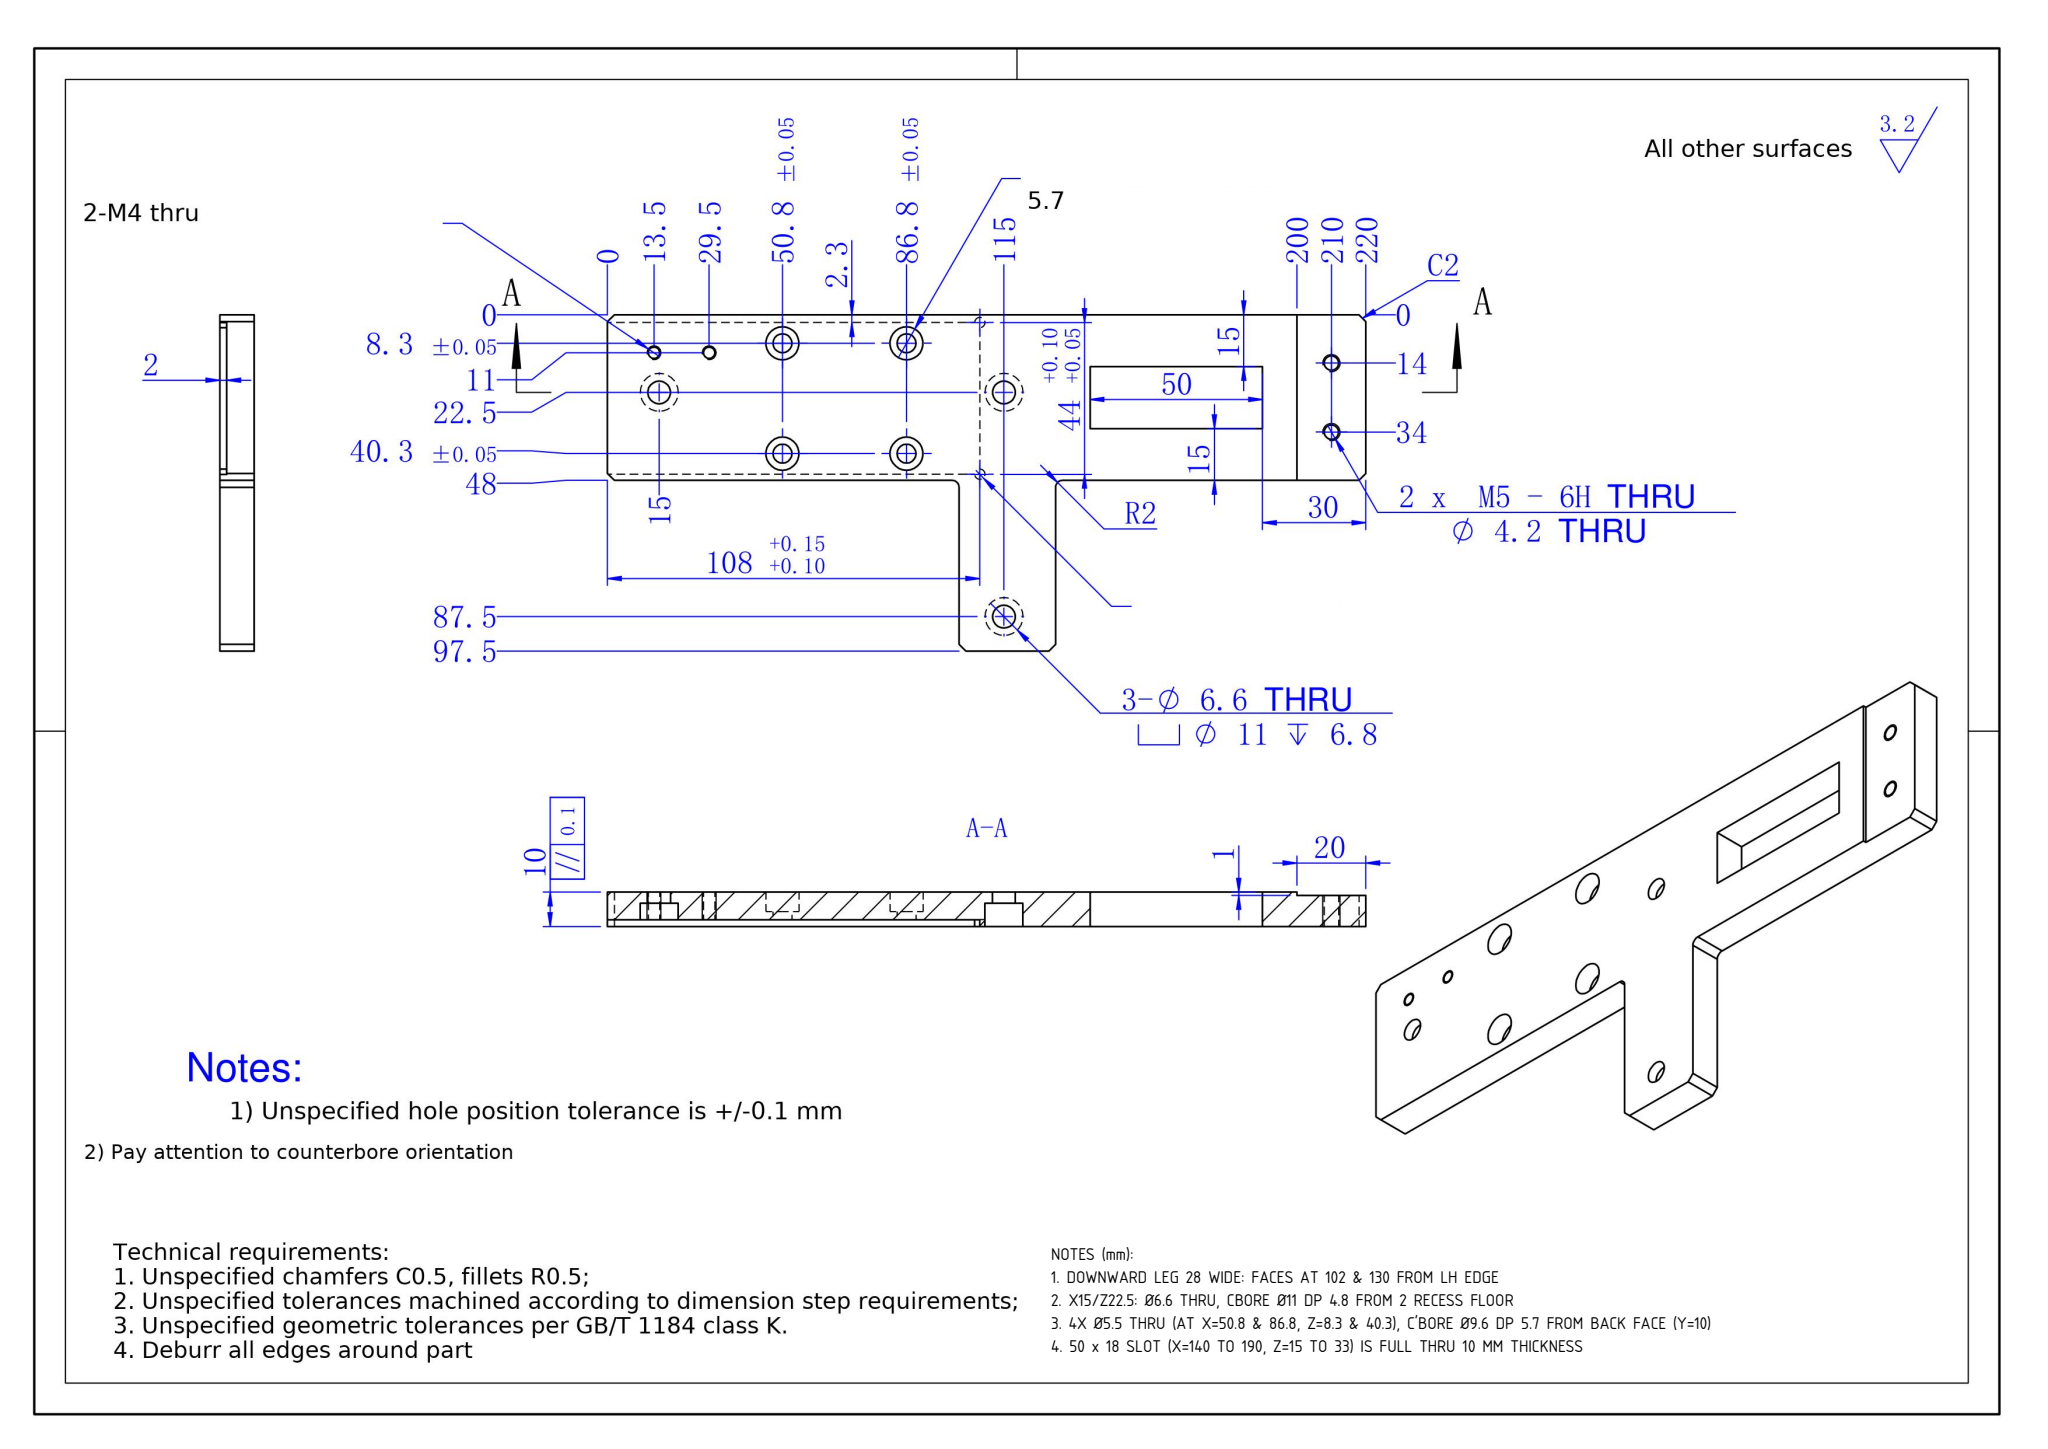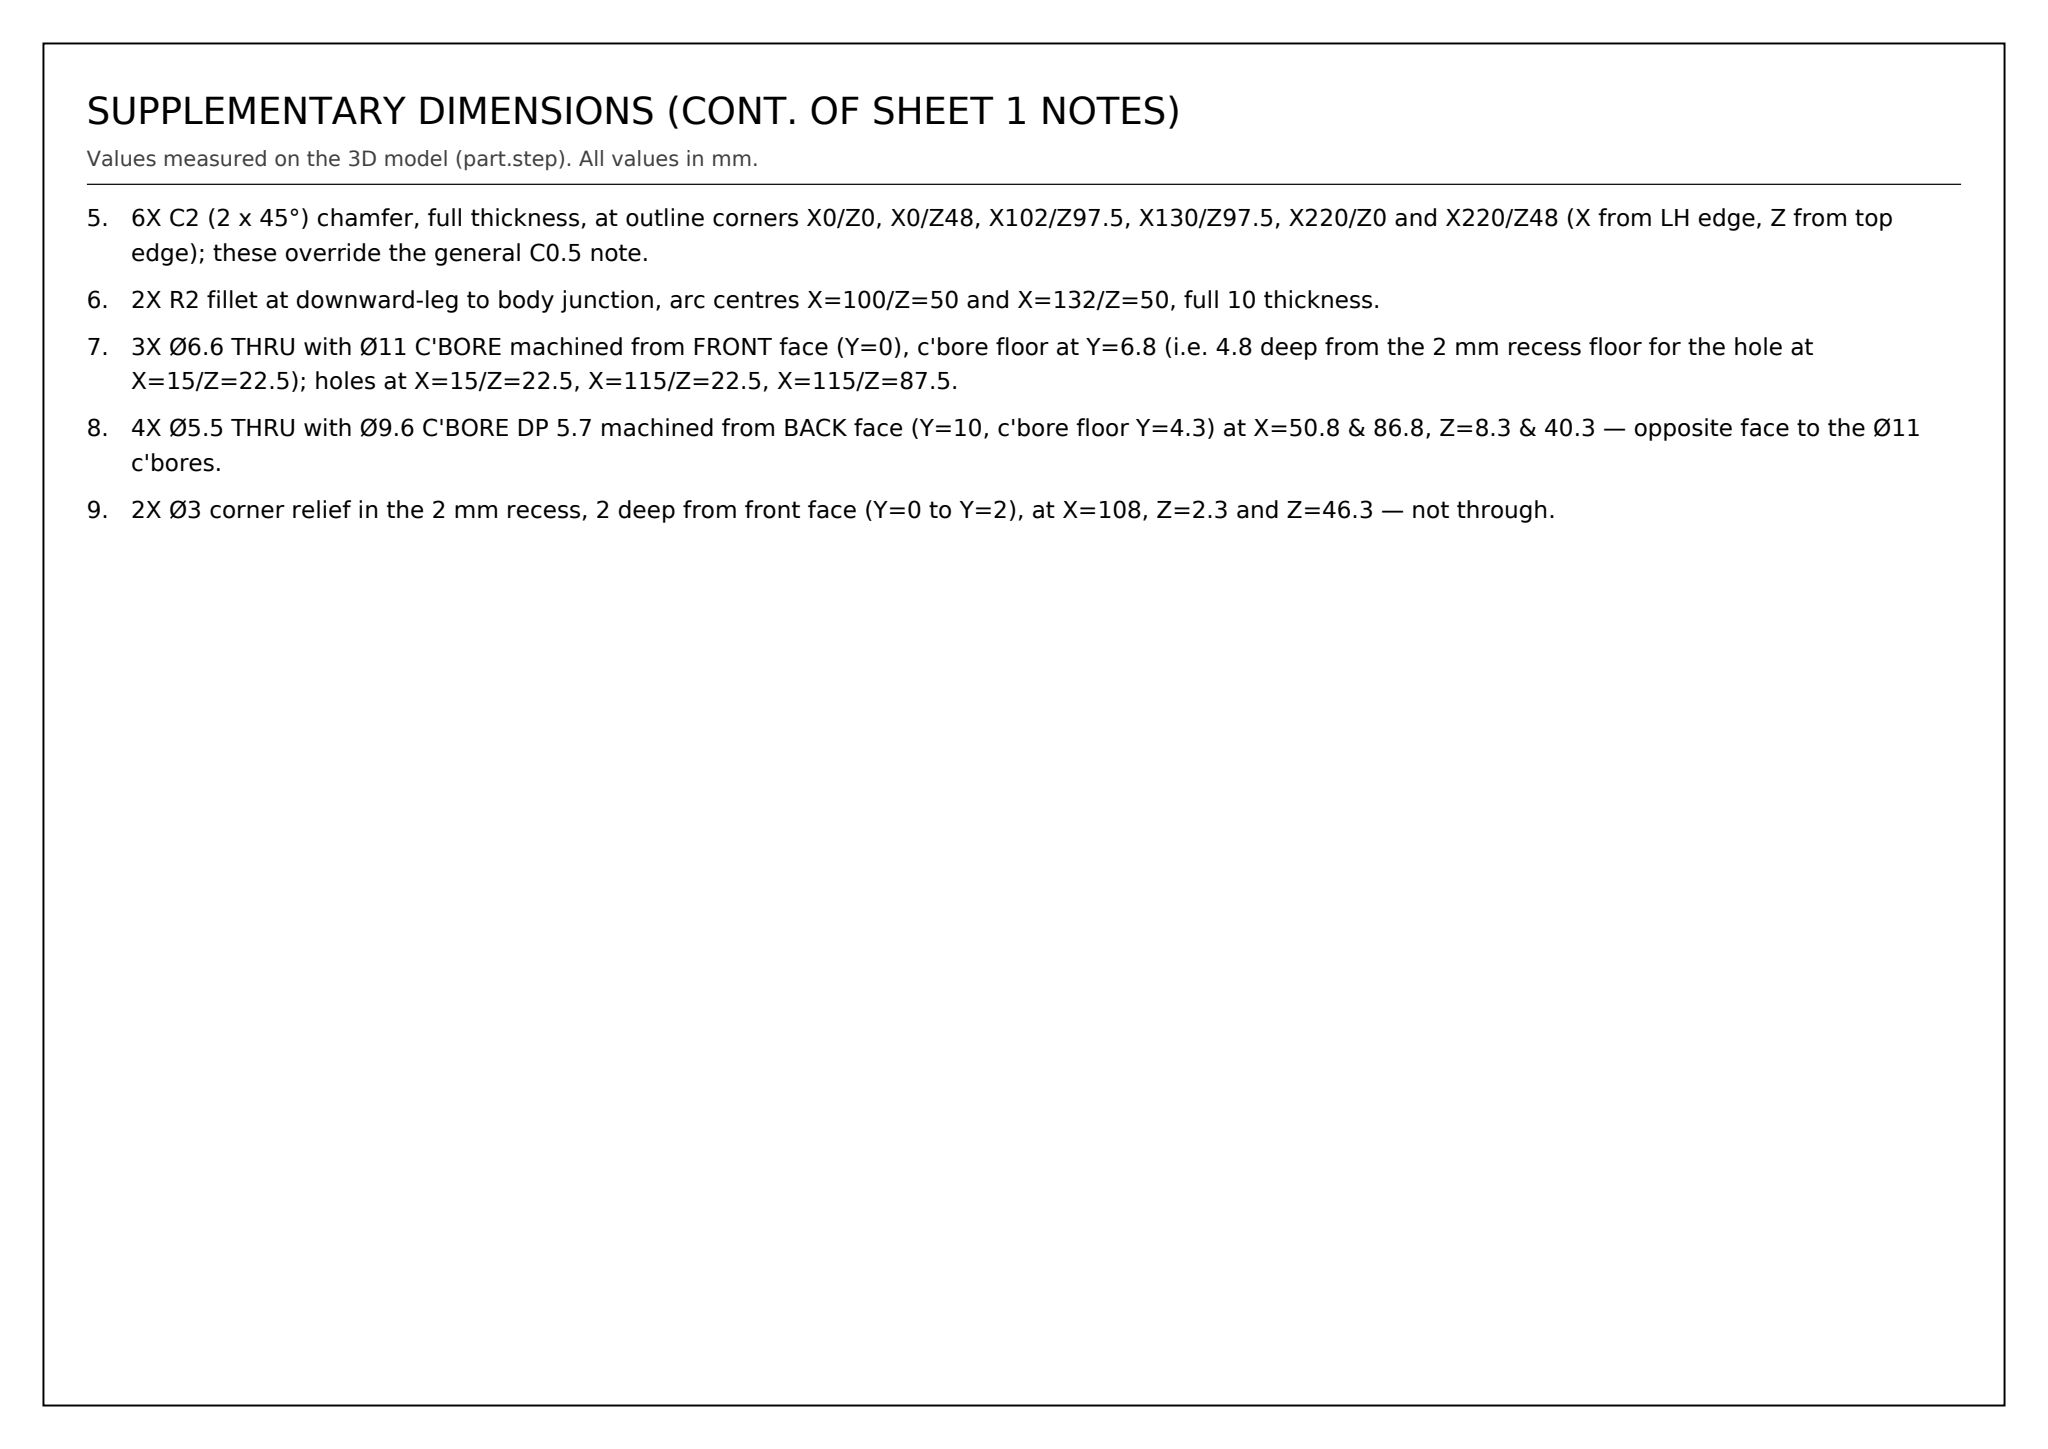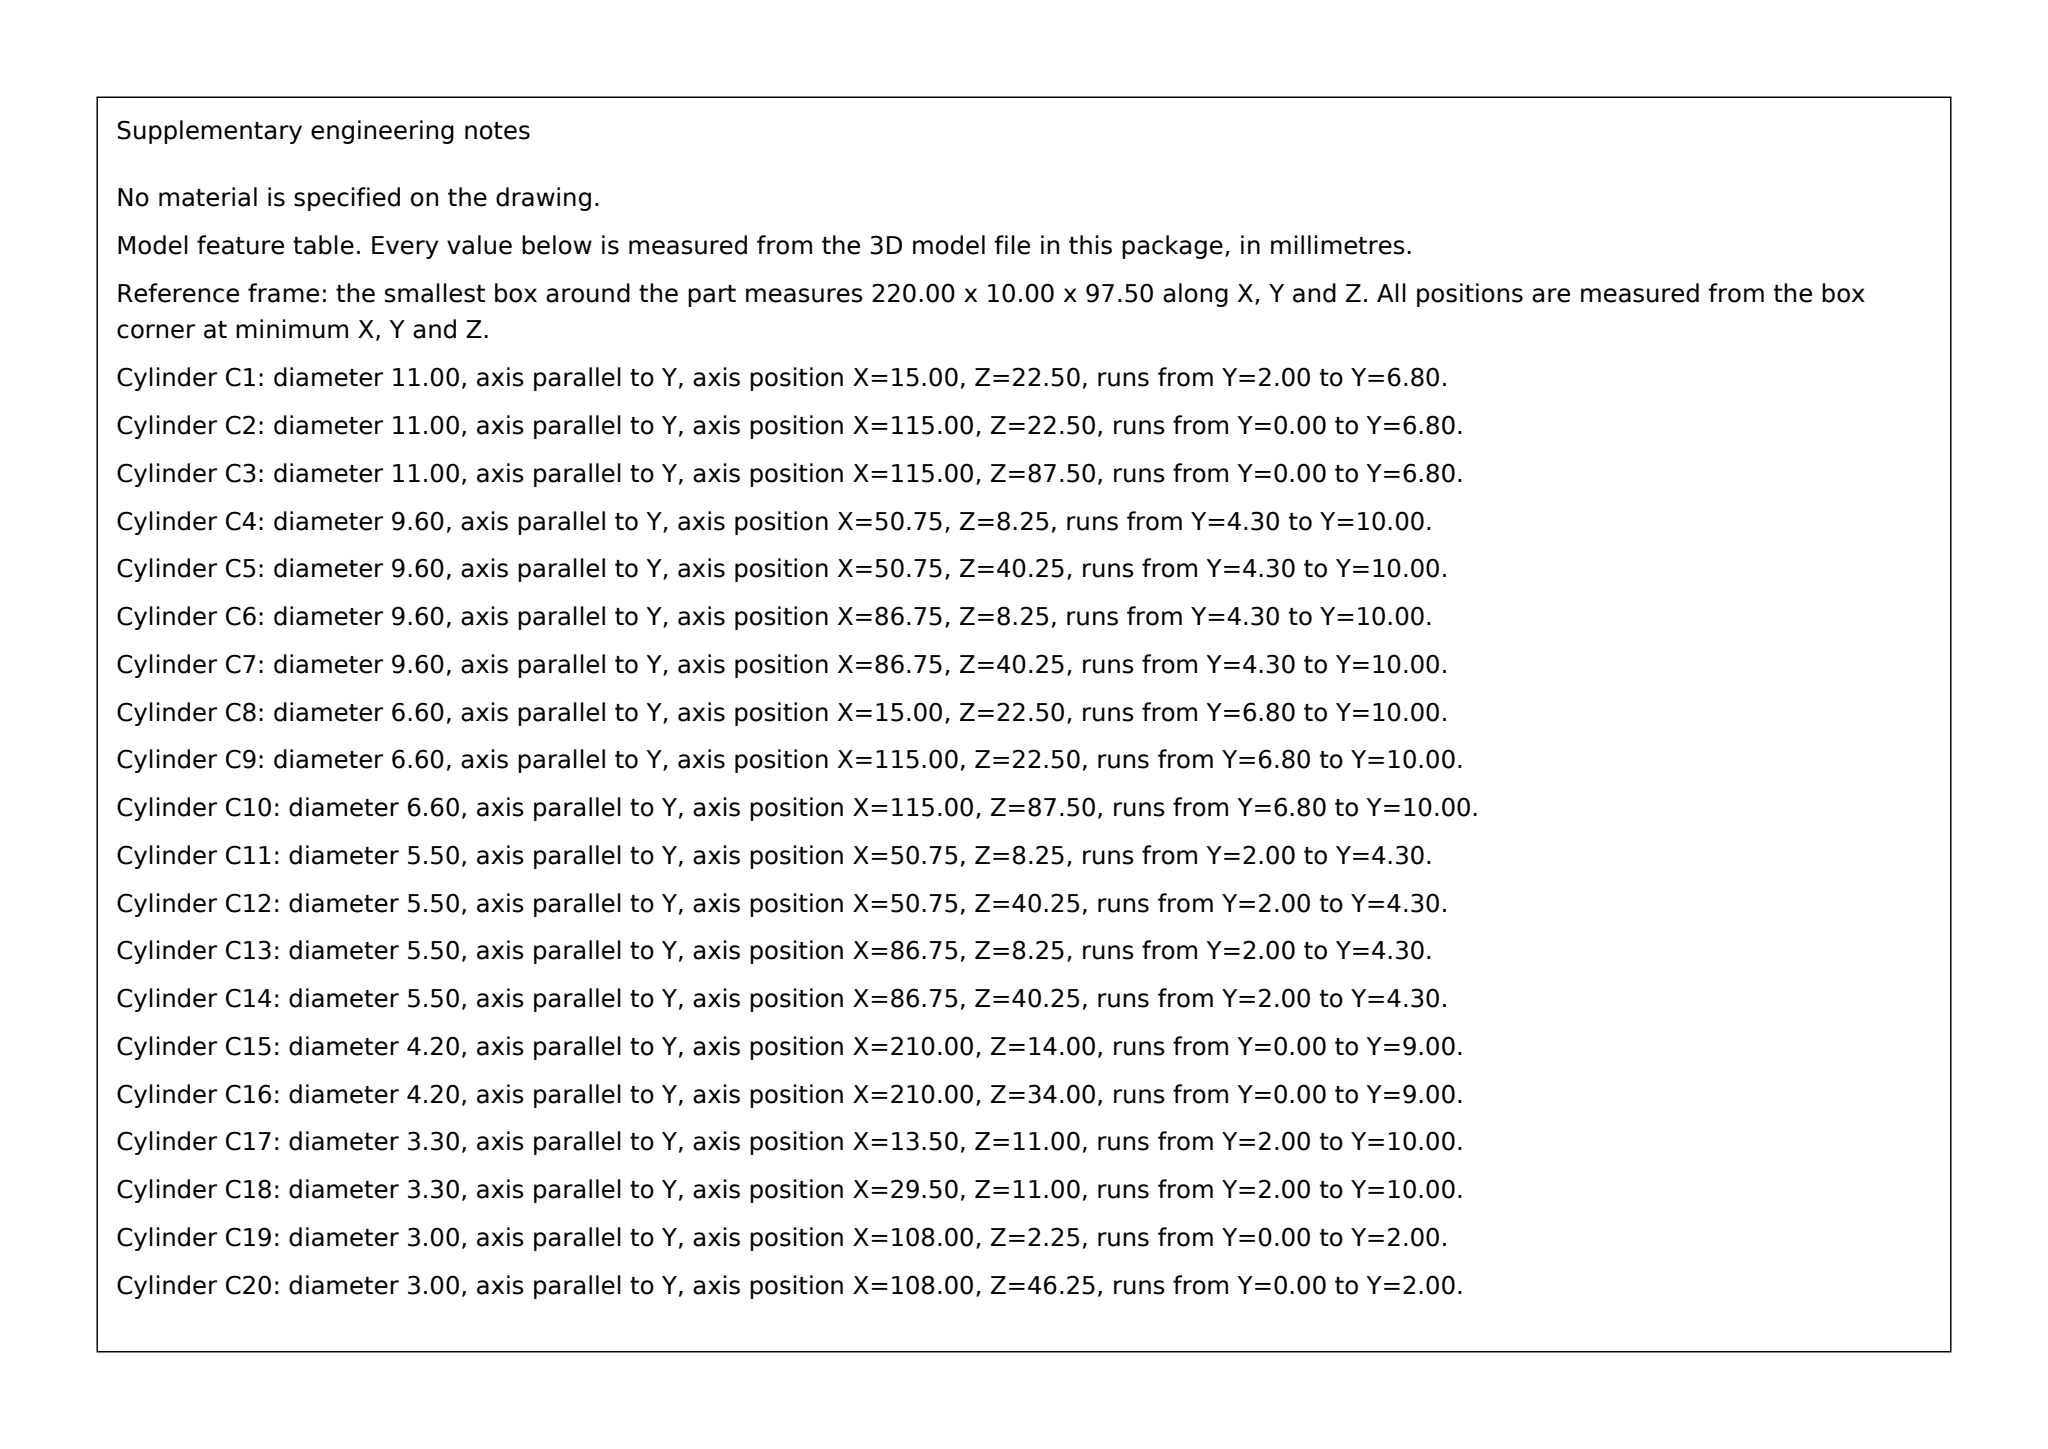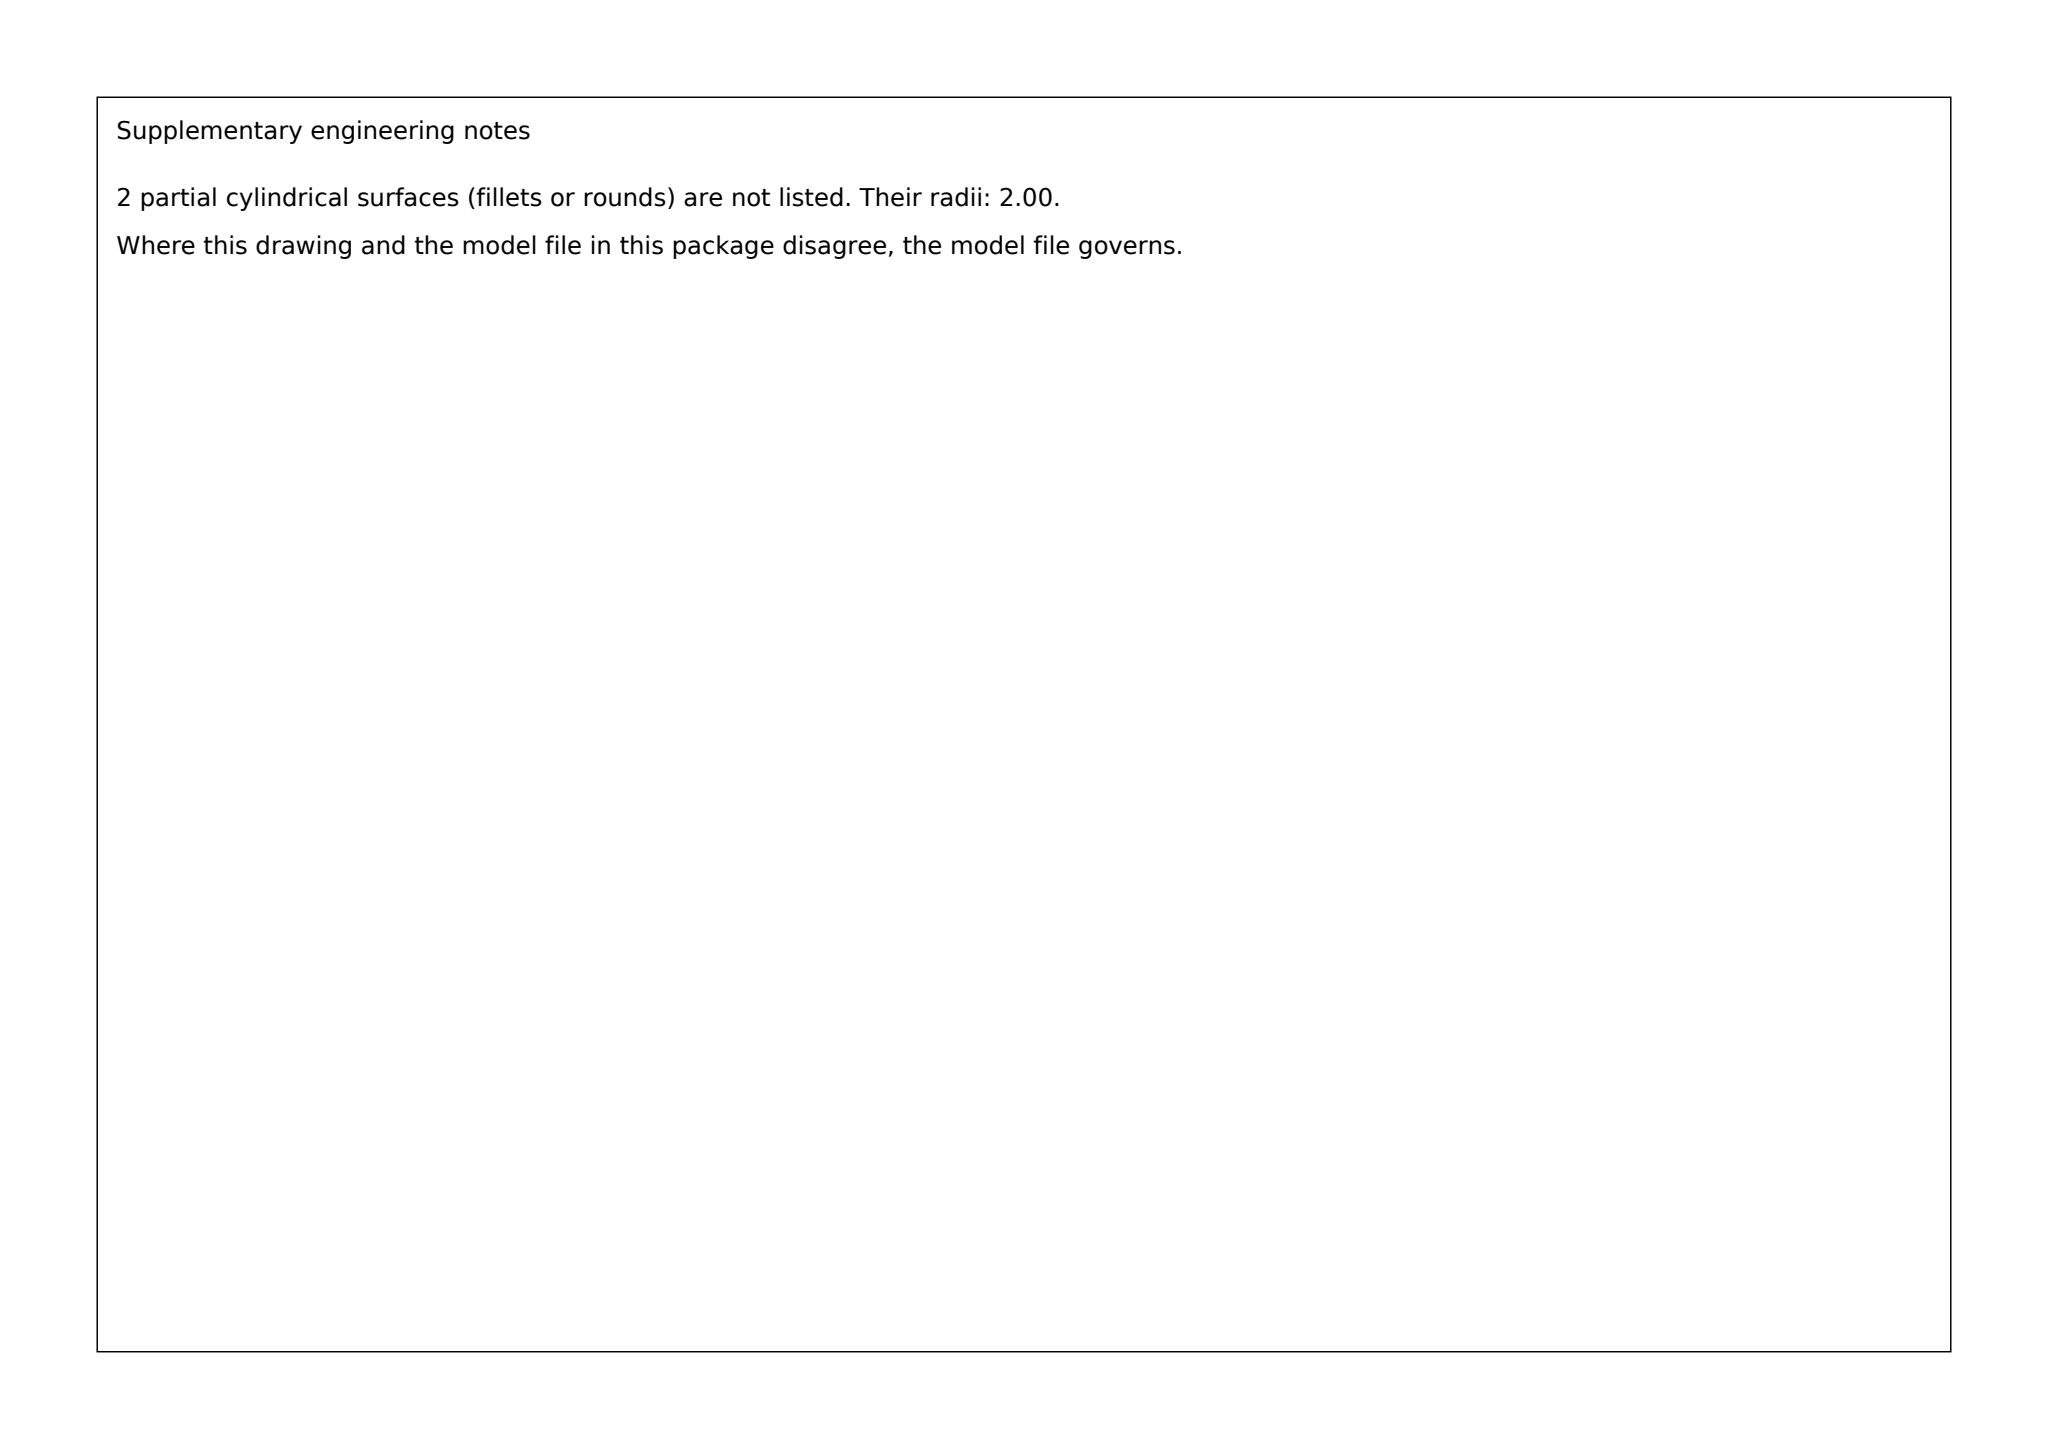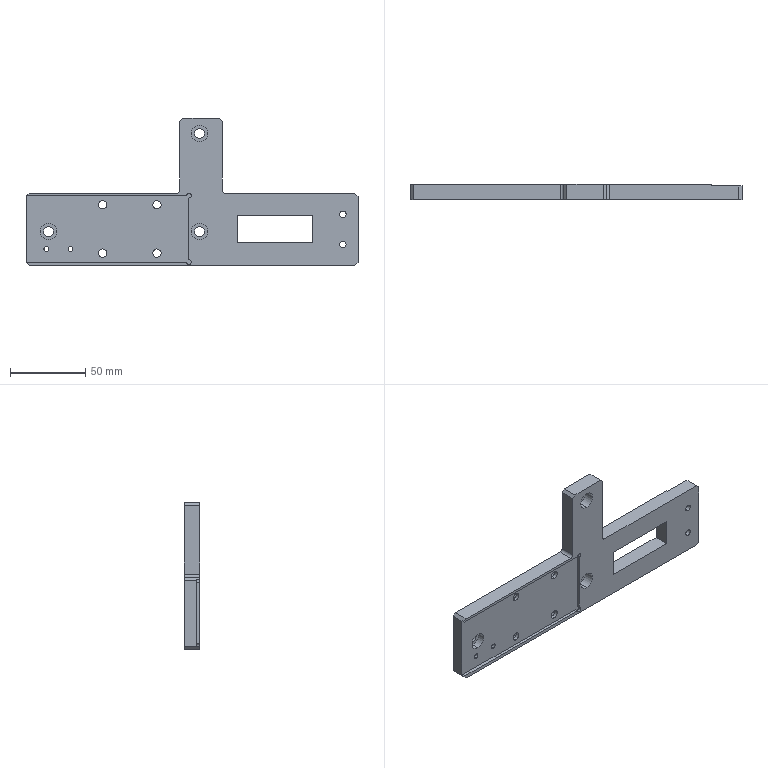Part | SolidWorks | mm | 1 solid | 74 faces | box 220 x 10 x 97.5 mm | volume 95544 mm3 | cylinder 41 | plane 33 | commonest cylinder face diameters 9.6 x8 5.5 x8 11 x6 6.6 x6 3.3 x4 4.2 x4 3 x3 4 x2
Drawing notes:
DOWNWARD LEG 28 WIDE: FACES AT 102 & 130 FROM LH EDGE | from the solid: x-planes at 102.0 and 130.0; 130-102 = 28; LH edge = x 0
X15/Z22.5: Ø6.6 THRU, CBORE Ø11 DP 4.8 FROM 2 RECESS FLOOR | from the solid: cylinders [6.6,'y',[15.0,null,22.5],3.2] and [11.0,'y',[15.0,null,22.5],4.8] vs 6.8 deep at X115 holes
4X Ø5.5 THRU (AT X=50.8 & 86.8, Z=8.3 & 40.3), C'BORE Ø9.6 DP 5.7 FROM BACK FACE (Y=10) | from the solid: cylinders: dia 5.5 axis y at [50.8/86.8, z 8.3/40.3] from 2.0 to 4.3; dia 9.6 same axes from 4.3 to 10.0
50 x 18 SLOT (X=140 TO 190, Z=15 TO 33) IS FULL THRU 10 MM THICKNESS | from the solid: axis_planes x=140 & x=190 extent y [0,10], z [15,33]; planes z=15 & z=33 extent y [0,10]
6X C2 (2 x 45°) chamfer, full thickness, at outline corners X0/Z0, X0/Z48, X102/Z97.5, X130/Z97.5, X220/Z0 and X220/Z48 (X from LH edge, Z from top edge); these override the general C0.5 note. | from the solid: inclined_planes: six 45° faces, size 2 x 10 x 2 (2 x 9 x 2 at X218), bbox_from [0,0,0], [0,0,46], [102,0,95.5], [128,0,95.5], [218,0,0], [218,0,46]
2X R2 fillet at downward-leg to body junction, arc centres X=100/Z=50 and X=132/Z=50, full 10 thickness. | from the solid: cylinders: concave arc dia 4.0, axis y at [100,-,50] and [132,-,50], from y=0 to y=10, arc 90°
3X Ø6.6 THRU with Ø11 C'BORE machined from FRONT face (Y=0), c'bore floor at Y=6.8 (i.e. 4.8 deep from the 2 mm recess floor for the hole at X=15/Z=22.5); holes at X=15/Z=22.5, X=115/Z=22.5, X=115/Z=87.5. | from the solid: cylinders: dia 11.0 axis y at [115,-,22.5] and [115,-,87.5] from y=0 to 6.8, at [15,-,22.5] from y=2.0 to 6.8; dia 6.6 from y=6.8 to 10.0
4X Ø5.5 THRU with Ø9.6 C'BORE DP 5.7 machined from BACK face (Y=10, c'bore floor Y=4.3) at X=50.8 & 86.8, Z=8.3 & 40.3 — opposite face to the Ø11 c'bores. | from the solid: cylinders: dia 9.6 axis y at [50.8/86.8, -, 8.3/40.3] from y=4.3 to 10.0; dia 5.5 same axes from y=2.0 to 4.3
2X Ø3 corner relief in the 2 mm recess, 2 deep from front face (Y=0 to Y=2), at X=108, Z=2.3 and Z=46.3 — not through. | from the solid: cylinders: concave arc dia 3.0, axis y at [108,-,2.3] and [108,-,46.3], from y=0 to y=2.0, arc 270°
build123d program:
from build123d import *

# Parameters (mm, degrees)
SKETCH1_W                                         = 130
SKETCH1_H                                         = 48
BOSS_EXTRUDE1_DEPTH                               = 10
HOLE_SIZE_ACCORDING_TO_HEXAGON_SOCKET_D           = 6.6
HOLE_SIZE_ACCORDING_TO_HEXAGON_SOCKET_CBORE_D     = 11
HOLE_SIZE_ACCORDING_TO_HEXAGON_SOCKET_CBORE_DEPTH = 6.8
SKETCH8_W                                         = 90
SKETCH8_H                                         = 48
BOSS_EXTRUDE2_DEPTH                               = 10
M5_TAPPED_HOLE1_D                                 = 4.2
CHAMFER1_SIZE                                     = 2
SKETCH12_W                                        = 28
SKETCH12_H                                        = 49.5
BOSS_EXTRUDE5_DEPTH                               = 10
HOLE_SIZE_ACCORDING_TO_HEXAGON_SOC_2_D            = 6.6
HOLE_SIZE_ACCORDING_TO_HEXAGON_SOC_2_CBORE_D      = 11
HOLE_SIZE_ACCORDING_TO_HEXAGON_SOC_2_CBORE_DEPTH  = 6.8
CHAMFER2_SIZE                                     = 2
FILLET1_R                                         = 2
SKETCH20_W                                        = 103.207
SKETCH20_H                                        = 82.705
CUT_EXTRUDE1_DEPTH                                = 1
HOLE_SIZE_ACCORDING_TO_HEXAGON_SOC_3_D            = 5.5
HOLE_SIZE_ACCORDING_TO_HEXAGON_SOC_3_CBORE_D      = 9.6
HOLE_SIZE_ACCORDING_TO_HEXAGON_SOC_3_CBORE_DEPTH  = 5.7
SKETCH23_W                                        = 44
SKETCH23_H                                        = 2
CUT_EXTRUDE7_DEPTH                                = 108
SIZE_MM_CLEARANCE_DOWEL_PIN_HOLE_1_D              = 3
SIZE_MM_CLEARANCE_DOWEL_PIN_HOLE_1_DEPTH          = 2
M4_TAPPED_HOLE1_D                                 = 3.3
SKETCH28_W                                        = 50
SKETCH28_H                                        = 18
CUT_EXTRUDE8_DEPTH                                = 42


with BuildPart() as part:
    # Sketch1 → Boss-Extrude1 (new body)
    with BuildSketch(Plane(origin=(0, 0, 0), x_dir=(1, 0, 0), z_dir=(0, 1, 0))):
        with Locations((65, 24)):
            Rectangle(SKETCH1_W, SKETCH1_H)
    extrude(amount=BOSS_EXTRUDE1_DEPTH)

    # Hole Size _According to_ Hexagon Socket (through all)
    with Locations(Plane(origin=(0, 0, 0), x_dir=(-1, 0, 0), z_dir=(0, -1, 0))):
        with Locations((-115, 25.5), (-15, 25.5)):
            CounterBoreHole(HOLE_SIZE_ACCORDING_TO_HEXAGON_SOCKET_D / 2, HOLE_SIZE_ACCORDING_TO_HEXAGON_SOCKET_CBORE_D / 2, HOLE_SIZE_ACCORDING_TO_HEXAGON_SOCKET_CBORE_DEPTH)

    # Sketch8 → Boss-Extrude2 (add)
    with BuildSketch(Plane(origin=(0, 10, 0), x_dir=(1, 0, 0), z_dir=(0, 1, 0))):
        with Locations((175, 24)):
            Rectangle(SKETCH8_W, SKETCH8_H)
    extrude(amount=-BOSS_EXTRUDE2_DEPTH)

    # M5 Tapped Hole1 (through all)
    with Locations(Plane(origin=(0, 10, 0), x_dir=(1, 0, 0), z_dir=(0, 1, 0))):
        with Locations((210, 34), (210, 14)):
            Hole(M5_TAPPED_HOLE1_D / 2)

    # Chamfer1
    chamfer1_edges = [part.edges().sort_by_distance(p)[0] for p in [
        (220, 5, -48),
        (220, 5, 0),
        (0, 5, -48),
        (0, 5, 0),
    ]]
    chamfer(chamfer1_edges, length=CHAMFER1_SIZE)

    # Sketch12 → Boss-Extrude5 (add)
    with BuildSketch(Plane.XZ):
        with Locations((116, 24.75)):
            Rectangle(SKETCH12_W, SKETCH12_H)
    extrude(amount=-BOSS_EXTRUDE5_DEPTH)

    # Hole Size _According to_ Hexagon Soc 2 (through all)
    with Locations(Plane(origin=(0, 0, 0), x_dir=(-1, 0, 0), z_dir=(0, -1, 0))):
        with Locations((-115, -39.5)):
            CounterBoreHole(HOLE_SIZE_ACCORDING_TO_HEXAGON_SOC_2_D / 2, HOLE_SIZE_ACCORDING_TO_HEXAGON_SOC_2_CBORE_D / 2, HOLE_SIZE_ACCORDING_TO_HEXAGON_SOC_2_CBORE_DEPTH)

    # Chamfer2
    chamfer2_edges = [part.edges().sort_by_distance(p)[0] for p in [
        (102, 5, 49.5),
        (130, 5, 49.5),
    ]]
    chamfer(chamfer2_edges, length=CHAMFER2_SIZE)

    # Fillet1
    fillet1_edges = [part.edges().sort_by_distance(p)[0] for p in [
        (102, 5, 0),
        (130, 5, 0),
    ]]
    fillet(fillet1_edges, radius=FILLET1_R)

    # Sketch20 → Cut-Extrude1 (cut)
    with BuildSketch(Plane(origin=(0, 10, 0), x_dir=(1, 0, 0), z_dir=(0, 1, 0))):
        with Locations((251.603, 22.152)):
            Rectangle(SKETCH20_W, SKETCH20_H)
    extrude(amount=-CUT_EXTRUDE1_DEPTH, mode=Mode.SUBTRACT)

    # Hole Size _According to_ Hexagon Soc 3 (through all)
    with Locations(Plane(origin=(0, 10, 0), x_dir=(1, 0, 0), z_dir=(0, 1, 0))):
        with Locations((50.75, 7.75), (86.75, 7.75), (50.75, 39.75), (86.75, 39.75)):
            CounterBoreHole(HOLE_SIZE_ACCORDING_TO_HEXAGON_SOC_3_D / 2, HOLE_SIZE_ACCORDING_TO_HEXAGON_SOC_3_CBORE_D / 2, HOLE_SIZE_ACCORDING_TO_HEXAGON_SOC_3_CBORE_DEPTH)

    # Sketch23 → Cut-Extrude7 (cut)
    with BuildSketch(Plane.ZY):
        with Locations((-23.75, 1)):
            Rectangle(SKETCH23_W, SKETCH23_H)
    extrude(amount=-CUT_EXTRUDE7_DEPTH, mode=Mode.SUBTRACT)

    # Size mm Clearance Dowel Pin Hole 1
    with Locations(Plane(origin=(0, 0, 0), x_dir=(-1, 0, 0), z_dir=(0, -1, 0))):
        with Locations((-108, 45.75), (-108, 1.75)):
            Hole(SIZE_MM_CLEARANCE_DOWEL_PIN_HOLE_1_D / 2, depth=SIZE_MM_CLEARANCE_DOWEL_PIN_HOLE_1_DEPTH)

    # M4 Tapped Hole1 (through all)
    with Locations(Plane(origin=(0, 10, 0), x_dir=(1, 0, 0), z_dir=(0, 1, 0))):
        with Locations((29.5, 37), (13.5, 37)):
            Hole(M4_TAPPED_HOLE1_D / 2)

    # Sketch28 → Cut-Extrude8 (cut)
    with BuildSketch(Plane.XZ):
        with Locations((165, -24)):
            Rectangle(SKETCH28_W, SKETCH28_H)
    extrude(amount=-CUT_EXTRUDE8_DEPTH, mode=Mode.SUBTRACT)


solid = part.part